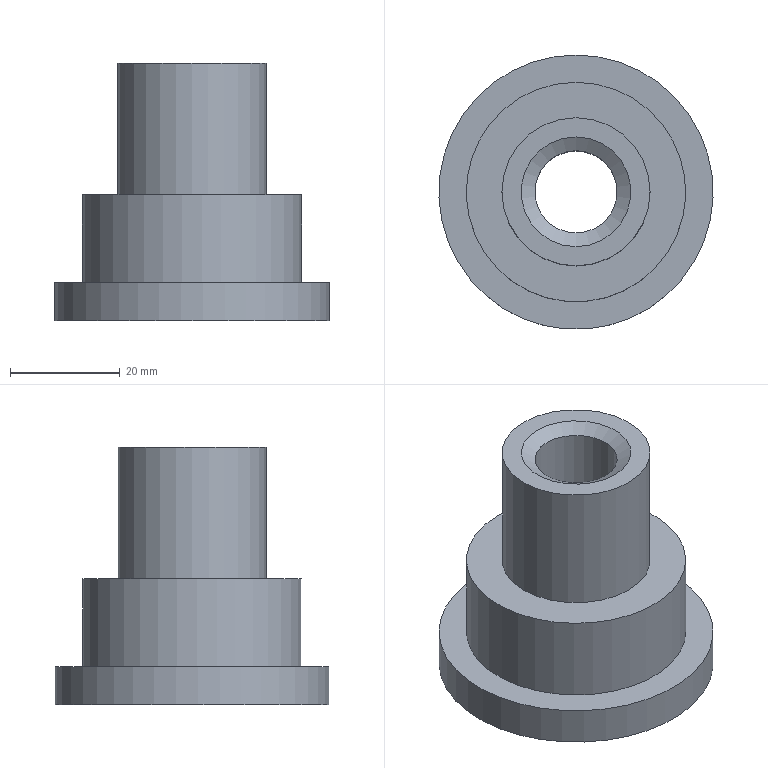Component | NX | BASE | 1 solid | 10 faces | box 50 x 50 x 47 mm | volume 38898 mm3 | cylinder 4 | plane 4 | cone 1 | torus 1 | commonest cylinder face diameters 15 x1 50 x1 40 x1 27 x1
STEP:
#1=CARTESIAN_POINT('',(0.,0.,0.));
#2=DIRECTION('',(0.,0.,1.));
#3=DIRECTION('',(1.,0.,0.));
#4=AXIS2_PLACEMENT_3D('',#1,#2,#3);
#5=CARTESIAN_POINT('',(-146.777,7.5,20.491));
#6=VERTEX_POINT('',#5);
#7=CARTESIAN_POINT('',(-146.777,0.,20.491));
#8=DIRECTION('',(0.,0.,-1.));
#9=DIRECTION('',(0.,1.,0.));
#10=AXIS2_PLACEMENT_3D('',#7,#8,#9);
#11=CIRCLE('',#10,7.5);
#12=CARTESIAN_POINT('',(-146.777,0.,22.491));
#13=DIRECTION('',(0.,0.,-1.));
#14=DIRECTION('',(0.,1.,0.));
#15=AXIS2_PLACEMENT_3D('',#12,#13,#14);
#16=CYLINDRICAL_SURFACE('',#15,7.5);
#17=CARTESIAN_POINT('',(0.,2.));
#18=DIRECTION('',(1.,0.));
#19=VECTOR('',#18,1.);
#20=LINE('',#17,#19);
#21=(GEOMETRIC_REPRESENTATION_CONTEXT(2)PARAMETRIC_REPRESENTATION_CONTEXT()REPRESENTATION_CONTEXT('',''));
#22=DEFINITIONAL_REPRESENTATION('',(#20),#21);
#23=PCURVE('',#16,#22);
#24=CARTESIAN_POINT('',(-146.777,0.,20.491));
#25=DIRECTION('',(0.,0.,-1.));
#26=DIRECTION('',(0.,1.,0.));
#27=AXIS2_PLACEMENT_3D('',#24,#25,#26);
#28=TOROIDAL_SURFACE('',#27,12.5,5.);
#29=CARTESIAN_POINT('',(0.,9.425));
#30=DIRECTION('',(1.,0.));
#31=VECTOR('',#30,1.);
#32=LINE('',#29,#31);
#33=(GEOMETRIC_REPRESENTATION_CONTEXT(2)PARAMETRIC_REPRESENTATION_CONTEXT()REPRESENTATION_CONTEXT('',''));
#34=DEFINITIONAL_REPRESENTATION('',(#32),#33);
#35=PCURVE('',#28,#34);
#36=SURFACE_CURVE('',#11,(#23,#35),.PCURVE_S1.);
#37=EDGE_CURVE('',#6,#6,#36,.T.);
#38=ORIENTED_EDGE('',*,*,#37,.F.);
#39=CARTESIAN_POINT('',(-146.777,7.5,60.991));
#40=VERTEX_POINT('',#39);
#41=CARTESIAN_POINT('',(-146.777,7.5,60.991));
#42=CARTESIAN_POINT('',(-146.777,7.5,20.491));
#43=B_SPLINE_CURVE_WITH_KNOTS('',1,(#41,#42),.UNSPECIFIED.,.F.,.F.,(2,2),(-38.5,2.),.PIECEWISE_BEZIER_KNOTS.);
#44=CARTESIAN_POINT('',(0.,0.));
#45=DIRECTION('',(0.,1.));
#46=VECTOR('',#45,1.);
#47=LINE('',#44,#46);
#48=(GEOMETRIC_REPRESENTATION_CONTEXT(2)PARAMETRIC_REPRESENTATION_CONTEXT()REPRESENTATION_CONTEXT('',''));
#49=DEFINITIONAL_REPRESENTATION('',(#47),#48);
#50=PCURVE('',#16,#49);
#51=CARTESIAN_POINT('',(6.283,0.));
#52=DIRECTION('',(0.,1.));
#53=VECTOR('',#52,1.);
#54=LINE('',#51,#53);
#55=(GEOMETRIC_REPRESENTATION_CONTEXT(2)PARAMETRIC_REPRESENTATION_CONTEXT()REPRESENTATION_CONTEXT('',''));
#56=DEFINITIONAL_REPRESENTATION('',(#54),#55);
#57=PCURVE('',#16,#56);
#58=SEAM_CURVE('',#43,(#50,#57),.PCURVE_S1.);
#59=EDGE_CURVE('',#40,#6,#58,.T.);
#60=ORIENTED_EDGE('',*,*,#59,.F.);
#61=CARTESIAN_POINT('',(-146.777,-7.5,60.991));
#62=VERTEX_POINT('',#61);
#63=CARTESIAN_POINT('',(-146.777,0.,60.991));
#64=DIRECTION('',(0.,0.,1.));
#65=DIRECTION('',(0.,-1.,0.));
#66=AXIS2_PLACEMENT_3D('',#63,#64,#65);
#67=CIRCLE('',#66,7.5);
#68=CARTESIAN_POINT('',(3.142,-38.5));
#69=DIRECTION('',(-1.,0.));
#70=VECTOR('',#69,1.);
#71=LINE('',#68,#70);
#72=(GEOMETRIC_REPRESENTATION_CONTEXT(2)PARAMETRIC_REPRESENTATION_CONTEXT()REPRESENTATION_CONTEXT('',''));
#73=DEFINITIONAL_REPRESENTATION('',(#71),#72);
#74=PCURVE('',#16,#73);
#75=CARTESIAN_POINT('',(-146.777,0.,62.491));
#76=DIRECTION('',(0.,0.,1.));
#77=DIRECTION('',(0.,-1.,0.));
#78=AXIS2_PLACEMENT_3D('',#75,#76,#77);
#79=CONICAL_SURFACE('',#78,10.,1.03);
#80=CARTESIAN_POINT('',(0.,-1.5));
#81=DIRECTION('',(1.,0.));
#82=VECTOR('',#81,1.);
#83=LINE('',#80,#82);
#84=(GEOMETRIC_REPRESENTATION_CONTEXT(2)PARAMETRIC_REPRESENTATION_CONTEXT()REPRESENTATION_CONTEXT('',''));
#85=DEFINITIONAL_REPRESENTATION('',(#83),#84);
#86=PCURVE('',#79,#85);
#87=SURFACE_CURVE('',#67,(#74,#86),.PCURVE_S1.);
#88=EDGE_CURVE('',#62,#40,#87,.T.);
#89=ORIENTED_EDGE('',*,*,#88,.F.);
#90=CARTESIAN_POINT('',(-146.777,0.,60.991));
#91=DIRECTION('',(0.,0.,1.));
#92=DIRECTION('',(0.,-1.,0.));
#93=AXIS2_PLACEMENT_3D('',#90,#91,#92);
#94=CIRCLE('',#93,7.5);
#95=CARTESIAN_POINT('',(9.425,-38.5));
#96=DIRECTION('',(-1.,0.));
#97=VECTOR('',#96,1.);
#98=LINE('',#95,#97);
#99=(GEOMETRIC_REPRESENTATION_CONTEXT(2)PARAMETRIC_REPRESENTATION_CONTEXT()REPRESENTATION_CONTEXT('',''));
#100=DEFINITIONAL_REPRESENTATION('',(#98),#99);
#101=PCURVE('',#16,#100);
#102=CARTESIAN_POINT('',(0.,-1.5));
#103=DIRECTION('',(1.,0.));
#104=VECTOR('',#103,1.);
#105=LINE('',#102,#104);
#106=(GEOMETRIC_REPRESENTATION_CONTEXT(2)PARAMETRIC_REPRESENTATION_CONTEXT()REPRESENTATION_CONTEXT('',''));
#107=DEFINITIONAL_REPRESENTATION('',(#105),#106);
#108=PCURVE('',#79,#107);
#109=SURFACE_CURVE('',#94,(#101,#108),.PCURVE_S1.);
#110=EDGE_CURVE('',#40,#62,#109,.T.);
#111=ORIENTED_EDGE('',*,*,#110,.F.);
#112=ORIENTED_EDGE('',*,*,#59,.T.);
#113=EDGE_LOOP('',(#38,#60,#89,#111,#112));
#114=FACE_BOUND('',#113,.F.);
#115=ADVANCED_FACE('',(#114),#16,.F.);
#116=CARTESIAN_POINT('',(-146.777,12.5,15.491));
#117=VERTEX_POINT('',#116);
#118=CARTESIAN_POINT('',(-146.777,0.,15.491));
#119=DIRECTION('',(0.,0.,1.));
#120=DIRECTION('',(0.,1.,0.));
#121=AXIS2_PLACEMENT_3D('',#118,#119,#120);
#122=CIRCLE('',#121,12.5);
#123=CARTESIAN_POINT('',(-139.277,0.,15.491));
#124=DIRECTION('',(0.,0.,-1.));
#125=DIRECTION('',(0.,1.,0.));
#126=AXIS2_PLACEMENT_3D('',#123,#124,#125);
#127=PLANE('',#126);
#128=CARTESIAN_POINT('',(12.5,-7.5));
#129=CARTESIAN_POINT('',(12.5,-29.151));
#130=CARTESIAN_POINT('',(-6.25,-18.325));
#131=CARTESIAN_POINT('',(-25.,-7.5));
#132=CARTESIAN_POINT('',(-6.25,3.325));
#133=CARTESIAN_POINT('',(12.5,14.151));
#134=CARTESIAN_POINT('',(12.5,-7.5));
#135=(BOUNDED_CURVE()B_SPLINE_CURVE(2,(#128,#129,#130,#131,#132,#133,#134),.UNSPECIFIED.,.T.,.F.)B_SPLINE_CURVE_WITH_KNOTS((1,2,2,2,2,1),(-2.094,0.,2.094,4.189,6.283,8.378),.UNSPECIFIED.)CURVE()GEOMETRIC_REPRESENTATION_ITEM()RATIONAL_B_SPLINE_CURVE((1.,0.5,1.,0.5,1.,0.5,1.))REPRESENTATION_ITEM(''));
#136=(GEOMETRIC_REPRESENTATION_CONTEXT(2)PARAMETRIC_REPRESENTATION_CONTEXT()REPRESENTATION_CONTEXT('',''));
#137=DEFINITIONAL_REPRESENTATION('',(#135),#136);
#138=PCURVE('',#127,#137);
#139=CARTESIAN_POINT('',(6.283,7.854));
#140=DIRECTION('',(-1.,0.));
#141=VECTOR('',#140,1.);
#142=LINE('',#139,#141);
#143=(GEOMETRIC_REPRESENTATION_CONTEXT(2)PARAMETRIC_REPRESENTATION_CONTEXT()REPRESENTATION_CONTEXT('',''));
#144=DEFINITIONAL_REPRESENTATION('',(#142),#143);
#145=PCURVE('',#28,#144);
#146=SURFACE_CURVE('',#122,(#138,#145),.PCURVE_S1.);
#147=EDGE_CURVE('',#117,#117,#146,.T.);
#148=ORIENTED_EDGE('',*,*,#147,.T.);
#149=EDGE_LOOP('',(#148));
#150=FACE_BOUND('',#149,.T.);
#151=CARTESIAN_POINT('',(-146.777,25.,15.491));
#152=VERTEX_POINT('',#151);
#153=CARTESIAN_POINT('',(-146.777,0.,15.491));
#154=DIRECTION('',(0.,0.,-1.));
#155=DIRECTION('',(0.,1.,0.));
#156=AXIS2_PLACEMENT_3D('',#153,#154,#155);
#157=CIRCLE('',#156,25.);
#158=CARTESIAN_POINT('',(0.,-7.5));
#159=DIRECTION('',(1.,0.));
#160=AXIS2_PLACEMENT_2D('',#158,#159);
#161=CIRCLE('',#160,25.);
#162=(GEOMETRIC_REPRESENTATION_CONTEXT(2)PARAMETRIC_REPRESENTATION_CONTEXT()REPRESENTATION_CONTEXT('',''));
#163=DEFINITIONAL_REPRESENTATION('',(#161),#162);
#164=PCURVE('',#127,#163);
#165=CARTESIAN_POINT('',(-146.777,0.,22.491));
#166=DIRECTION('',(0.,0.,-1.));
#167=DIRECTION('',(0.,1.,0.));
#168=AXIS2_PLACEMENT_3D('',#165,#166,#167);
#169=CYLINDRICAL_SURFACE('',#168,25.);
#170=CARTESIAN_POINT('',(0.,7.));
#171=DIRECTION('',(1.,0.));
#172=VECTOR('',#171,1.);
#173=LINE('',#170,#172);
#174=(GEOMETRIC_REPRESENTATION_CONTEXT(2)PARAMETRIC_REPRESENTATION_CONTEXT()REPRESENTATION_CONTEXT('',''));
#175=DEFINITIONAL_REPRESENTATION('',(#173),#174);
#176=PCURVE('',#169,#175);
#177=SURFACE_CURVE('',#157,(#164,#176),.PCURVE_S1.);
#178=EDGE_CURVE('',#152,#152,#177,.T.);
#179=ORIENTED_EDGE('',*,*,#178,.T.);
#180=EDGE_LOOP('',(#179));
#181=FACE_BOUND('',#180,.T.);
#182=ADVANCED_FACE('',(#150,#181),#127,.T.);
#183=CARTESIAN_POINT('',(-146.777,25.,22.491));
#184=VERTEX_POINT('',#183);
#185=CARTESIAN_POINT('',(-146.777,0.,22.491));
#186=DIRECTION('',(0.,0.,-1.));
#187=DIRECTION('',(0.,1.,0.));
#188=AXIS2_PLACEMENT_3D('',#185,#186,#187);
#189=CIRCLE('',#188,25.);
#190=CARTESIAN_POINT('',(0.,0.));
#191=DIRECTION('',(1.,0.));
#192=VECTOR('',#191,1.);
#193=LINE('',#190,#192);
#194=(GEOMETRIC_REPRESENTATION_CONTEXT(2)PARAMETRIC_REPRESENTATION_CONTEXT()REPRESENTATION_CONTEXT('',''));
#195=DEFINITIONAL_REPRESENTATION('',(#193),#194);
#196=PCURVE('',#169,#195);
#197=CARTESIAN_POINT('',(-121.777,0.,22.491));
#198=DIRECTION('',(0.,0.,1.));
#199=DIRECTION('',(0.,-1.,0.));
#200=AXIS2_PLACEMENT_3D('',#197,#198,#199);
#201=PLANE('',#200);
#202=CARTESIAN_POINT('',(-25.,-25.));
#203=CARTESIAN_POINT('',(-25.,18.301));
#204=CARTESIAN_POINT('',(12.5,-3.349));
#205=CARTESIAN_POINT('',(50.,-25.));
#206=CARTESIAN_POINT('',(12.5,-46.651));
#207=CARTESIAN_POINT('',(-25.,-68.301));
#208=CARTESIAN_POINT('',(-25.,-25.));
#209=(BOUNDED_CURVE()B_SPLINE_CURVE(2,(#202,#203,#204,#205,#206,#207,#208),.UNSPECIFIED.,.T.,.F.)B_SPLINE_CURVE_WITH_KNOTS((1,2,2,2,2,1),(-2.094,0.,2.094,4.189,6.283,8.378),.UNSPECIFIED.)CURVE()GEOMETRIC_REPRESENTATION_ITEM()RATIONAL_B_SPLINE_CURVE((1.,0.5,1.,0.5,1.,0.5,1.))REPRESENTATION_ITEM(''));
#210=(GEOMETRIC_REPRESENTATION_CONTEXT(2)PARAMETRIC_REPRESENTATION_CONTEXT()REPRESENTATION_CONTEXT('',''));
#211=DEFINITIONAL_REPRESENTATION('',(#209),#210);
#212=PCURVE('',#201,#211);
#213=SURFACE_CURVE('',#189,(#196,#212),.PCURVE_S1.);
#214=EDGE_CURVE('',#184,#184,#213,.T.);
#215=ORIENTED_EDGE('',*,*,#214,.T.);
#216=CARTESIAN_POINT('',(-146.777,25.,22.491));
#217=CARTESIAN_POINT('',(-146.777,25.,15.491));
#218=B_SPLINE_CURVE_WITH_KNOTS('',1,(#216,#217),.UNSPECIFIED.,.F.,.F.,(2,2),(0.,7.),.PIECEWISE_BEZIER_KNOTS.);
#219=CARTESIAN_POINT('',(6.283,0.));
#220=DIRECTION('',(0.,1.));
#221=VECTOR('',#220,1.);
#222=LINE('',#219,#221);
#223=(GEOMETRIC_REPRESENTATION_CONTEXT(2)PARAMETRIC_REPRESENTATION_CONTEXT()REPRESENTATION_CONTEXT('',''));
#224=DEFINITIONAL_REPRESENTATION('',(#222),#223);
#225=PCURVE('',#169,#224);
#226=CARTESIAN_POINT('',(0.,0.));
#227=DIRECTION('',(0.,1.));
#228=VECTOR('',#227,1.);
#229=LINE('',#226,#228);
#230=(GEOMETRIC_REPRESENTATION_CONTEXT(2)PARAMETRIC_REPRESENTATION_CONTEXT()REPRESENTATION_CONTEXT('',''));
#231=DEFINITIONAL_REPRESENTATION('',(#229),#230);
#232=PCURVE('',#169,#231);
#233=SEAM_CURVE('',#218,(#225,#232),.PCURVE_S1.);
#234=EDGE_CURVE('',#184,#152,#233,.T.);
#235=ORIENTED_EDGE('',*,*,#234,.T.);
#236=ORIENTED_EDGE('',*,*,#178,.F.);
#237=ORIENTED_EDGE('',*,*,#234,.F.);
#238=EDGE_LOOP('',(#215,#235,#236,#237));
#239=FACE_BOUND('',#238,.T.);
#240=ADVANCED_FACE('',(#239),#169,.T.);
#241=CARTESIAN_POINT('',(-146.777,20.,22.491));
#242=VERTEX_POINT('',#241);
#243=CARTESIAN_POINT('',(-146.777,0.,22.491));
#244=DIRECTION('',(0.,0.,-1.));
#245=DIRECTION('',(0.,1.,0.));
#246=AXIS2_PLACEMENT_3D('',#243,#244,#245);
#247=CIRCLE('',#246,20.);
#248=CARTESIAN_POINT('',(-20.,-25.));
#249=CARTESIAN_POINT('',(-20.,9.641));
#250=CARTESIAN_POINT('',(10.,-7.679));
#251=CARTESIAN_POINT('',(40.,-25.));
#252=CARTESIAN_POINT('',(10.,-42.321));
#253=CARTESIAN_POINT('',(-20.,-59.641));
#254=CARTESIAN_POINT('',(-20.,-25.));
#255=(BOUNDED_CURVE()B_SPLINE_CURVE(2,(#248,#249,#250,#251,#252,#253,#254),.UNSPECIFIED.,.T.,.F.)B_SPLINE_CURVE_WITH_KNOTS((1,2,2,2,2,1),(-2.094,0.,2.094,4.189,6.283,8.378),.UNSPECIFIED.)CURVE()GEOMETRIC_REPRESENTATION_ITEM()RATIONAL_B_SPLINE_CURVE((1.,0.5,1.,0.5,1.,0.5,1.))REPRESENTATION_ITEM(''));
#256=(GEOMETRIC_REPRESENTATION_CONTEXT(2)PARAMETRIC_REPRESENTATION_CONTEXT()REPRESENTATION_CONTEXT('',''));
#257=DEFINITIONAL_REPRESENTATION('',(#255),#256);
#258=PCURVE('',#201,#257);
#259=CARTESIAN_POINT('',(-146.777,0.,22.491));
#260=DIRECTION('',(0.,0.,-1.));
#261=DIRECTION('',(0.,1.,0.));
#262=AXIS2_PLACEMENT_3D('',#259,#260,#261);
#263=CYLINDRICAL_SURFACE('',#262,20.);
#264=CARTESIAN_POINT('',(0.,0.));
#265=DIRECTION('',(1.,0.));
#266=VECTOR('',#265,1.);
#267=LINE('',#264,#266);
#268=(GEOMETRIC_REPRESENTATION_CONTEXT(2)PARAMETRIC_REPRESENTATION_CONTEXT()REPRESENTATION_CONTEXT('',''));
#269=DEFINITIONAL_REPRESENTATION('',(#267),#268);
#270=PCURVE('',#263,#269);
#271=SURFACE_CURVE('',#247,(#258,#270),.PCURVE_S1.);
#272=EDGE_CURVE('',#242,#242,#271,.T.);
#273=ORIENTED_EDGE('',*,*,#272,.T.);
#274=EDGE_LOOP('',(#273));
#275=FACE_BOUND('',#274,.T.);
#276=ORIENTED_EDGE('',*,*,#214,.F.);
#277=EDGE_LOOP('',(#276));
#278=FACE_BOUND('',#277,.T.);
#279=ADVANCED_FACE('',(#275,#278),#201,.T.);
#280=CARTESIAN_POINT('',(-146.777,20.,38.491));
#281=VERTEX_POINT('',#280);
#282=CARTESIAN_POINT('',(-146.777,0.,38.491));
#283=DIRECTION('',(0.,0.,-1.));
#284=DIRECTION('',(0.,1.,0.));
#285=AXIS2_PLACEMENT_3D('',#282,#283,#284);
#286=CIRCLE('',#285,20.);
#287=CARTESIAN_POINT('',(0.,-16.));
#288=DIRECTION('',(1.,0.));
#289=VECTOR('',#288,1.);
#290=LINE('',#287,#289);
#291=(GEOMETRIC_REPRESENTATION_CONTEXT(2)PARAMETRIC_REPRESENTATION_CONTEXT()REPRESENTATION_CONTEXT('',''));
#292=DEFINITIONAL_REPRESENTATION('',(#290),#291);
#293=PCURVE('',#263,#292);
#294=CARTESIAN_POINT('',(-126.777,0.,38.491));
#295=DIRECTION('',(0.,0.,1.));
#296=DIRECTION('',(0.,-1.,0.));
#297=AXIS2_PLACEMENT_3D('',#294,#295,#296);
#298=PLANE('',#297);
#299=CARTESIAN_POINT('',(-20.,-20.));
#300=CARTESIAN_POINT('',(-20.,14.641));
#301=CARTESIAN_POINT('',(10.,-2.679));
#302=CARTESIAN_POINT('',(40.,-20.));
#303=CARTESIAN_POINT('',(10.,-37.321));
#304=CARTESIAN_POINT('',(-20.,-54.641));
#305=CARTESIAN_POINT('',(-20.,-20.));
#306=(BOUNDED_CURVE()B_SPLINE_CURVE(2,(#299,#300,#301,#302,#303,#304,#305),.UNSPECIFIED.,.T.,.F.)B_SPLINE_CURVE_WITH_KNOTS((1,2,2,2,2,1),(-2.094,0.,2.094,4.189,6.283,8.378),.UNSPECIFIED.)CURVE()GEOMETRIC_REPRESENTATION_ITEM()RATIONAL_B_SPLINE_CURVE((1.,0.5,1.,0.5,1.,0.5,1.))REPRESENTATION_ITEM(''));
#307=(GEOMETRIC_REPRESENTATION_CONTEXT(2)PARAMETRIC_REPRESENTATION_CONTEXT()REPRESENTATION_CONTEXT('',''));
#308=DEFINITIONAL_REPRESENTATION('',(#306),#307);
#309=PCURVE('',#298,#308);
#310=SURFACE_CURVE('',#286,(#293,#309),.PCURVE_S1.);
#311=EDGE_CURVE('',#281,#281,#310,.T.);
#312=ORIENTED_EDGE('',*,*,#311,.T.);
#313=CARTESIAN_POINT('',(-146.777,20.,38.491));
#314=CARTESIAN_POINT('',(-146.777,20.,22.491));
#315=B_SPLINE_CURVE_WITH_KNOTS('',1,(#313,#314),.UNSPECIFIED.,.F.,.F.,(2,2),(-16.,0.),.PIECEWISE_BEZIER_KNOTS.);
#316=CARTESIAN_POINT('',(6.283,0.));
#317=DIRECTION('',(0.,1.));
#318=VECTOR('',#317,1.);
#319=LINE('',#316,#318);
#320=(GEOMETRIC_REPRESENTATION_CONTEXT(2)PARAMETRIC_REPRESENTATION_CONTEXT()REPRESENTATION_CONTEXT('',''));
#321=DEFINITIONAL_REPRESENTATION('',(#319),#320);
#322=PCURVE('',#263,#321);
#323=CARTESIAN_POINT('',(0.,0.));
#324=DIRECTION('',(0.,1.));
#325=VECTOR('',#324,1.);
#326=LINE('',#323,#325);
#327=(GEOMETRIC_REPRESENTATION_CONTEXT(2)PARAMETRIC_REPRESENTATION_CONTEXT()REPRESENTATION_CONTEXT('',''));
#328=DEFINITIONAL_REPRESENTATION('',(#326),#327);
#329=PCURVE('',#263,#328);
#330=SEAM_CURVE('',#315,(#322,#329),.PCURVE_S1.);
#331=EDGE_CURVE('',#281,#242,#330,.T.);
#332=ORIENTED_EDGE('',*,*,#331,.T.);
#333=ORIENTED_EDGE('',*,*,#272,.F.);
#334=ORIENTED_EDGE('',*,*,#331,.F.);
#335=EDGE_LOOP('',(#312,#332,#333,#334));
#336=FACE_BOUND('',#335,.T.);
#337=ADVANCED_FACE('',(#336),#263,.T.);
#338=CARTESIAN_POINT('',(-146.777,13.5,38.491));
#339=VERTEX_POINT('',#338);
#340=CARTESIAN_POINT('',(-146.777,0.,38.491));
#341=DIRECTION('',(0.,0.,-1.));
#342=DIRECTION('',(0.,1.,0.));
#343=AXIS2_PLACEMENT_3D('',#340,#341,#342);
#344=CIRCLE('',#343,13.5);
#345=CARTESIAN_POINT('',(-13.5,-20.));
#346=CARTESIAN_POINT('',(-13.5,3.383));
#347=CARTESIAN_POINT('',(6.75,-8.309));
#348=CARTESIAN_POINT('',(27.,-20.));
#349=CARTESIAN_POINT('',(6.75,-31.691));
#350=CARTESIAN_POINT('',(-13.5,-43.383));
#351=CARTESIAN_POINT('',(-13.5,-20.));
#352=(BOUNDED_CURVE()B_SPLINE_CURVE(2,(#345,#346,#347,#348,#349,#350,#351),.UNSPECIFIED.,.T.,.F.)B_SPLINE_CURVE_WITH_KNOTS((1,2,2,2,2,1),(-2.094,0.,2.094,4.189,6.283,8.378),.UNSPECIFIED.)CURVE()GEOMETRIC_REPRESENTATION_ITEM()RATIONAL_B_SPLINE_CURVE((1.,0.5,1.,0.5,1.,0.5,1.))REPRESENTATION_ITEM(''));
#353=(GEOMETRIC_REPRESENTATION_CONTEXT(2)PARAMETRIC_REPRESENTATION_CONTEXT()REPRESENTATION_CONTEXT('',''));
#354=DEFINITIONAL_REPRESENTATION('',(#352),#353);
#355=PCURVE('',#298,#354);
#356=CARTESIAN_POINT('',(-146.777,0.,22.491));
#357=DIRECTION('',(0.,0.,-1.));
#358=DIRECTION('',(0.,1.,0.));
#359=AXIS2_PLACEMENT_3D('',#356,#357,#358);
#360=CYLINDRICAL_SURFACE('',#359,13.5);
#361=CARTESIAN_POINT('',(0.,-16.));
#362=DIRECTION('',(1.,0.));
#363=VECTOR('',#362,1.);
#364=LINE('',#361,#363);
#365=(GEOMETRIC_REPRESENTATION_CONTEXT(2)PARAMETRIC_REPRESENTATION_CONTEXT()REPRESENTATION_CONTEXT('',''));
#366=DEFINITIONAL_REPRESENTATION('',(#364),#365);
#367=PCURVE('',#360,#366);
#368=SURFACE_CURVE('',#344,(#355,#367),.PCURVE_S1.);
#369=EDGE_CURVE('',#339,#339,#368,.T.);
#370=ORIENTED_EDGE('',*,*,#369,.T.);
#371=EDGE_LOOP('',(#370));
#372=FACE_BOUND('',#371,.T.);
#373=ORIENTED_EDGE('',*,*,#311,.F.);
#374=EDGE_LOOP('',(#373));
#375=FACE_BOUND('',#374,.T.);
#376=ADVANCED_FACE('',(#372,#375),#298,.T.);
#377=CARTESIAN_POINT('',(-146.777,13.5,62.491));
#378=VERTEX_POINT('',#377);
#379=CARTESIAN_POINT('',(-146.777,0.,62.491));
#380=DIRECTION('',(0.,0.,-1.));
#381=DIRECTION('',(0.,1.,0.));
#382=AXIS2_PLACEMENT_3D('',#379,#380,#381);
#383=CIRCLE('',#382,13.5);
#384=CARTESIAN_POINT('',(0.,-40.));
#385=DIRECTION('',(1.,0.));
#386=VECTOR('',#385,1.);
#387=LINE('',#384,#386);
#388=(GEOMETRIC_REPRESENTATION_CONTEXT(2)PARAMETRIC_REPRESENTATION_CONTEXT()REPRESENTATION_CONTEXT('',''));
#389=DEFINITIONAL_REPRESENTATION('',(#387),#388);
#390=PCURVE('',#360,#389);
#391=CARTESIAN_POINT('',(-133.277,0.,62.491));
#392=DIRECTION('',(0.,0.,1.));
#393=DIRECTION('',(0.,-1.,0.));
#394=AXIS2_PLACEMENT_3D('',#391,#392,#393);
#395=PLANE('',#394);
#396=CARTESIAN_POINT('',(-13.5,-13.5));
#397=CARTESIAN_POINT('',(-13.5,9.883));
#398=CARTESIAN_POINT('',(6.75,-1.809));
#399=CARTESIAN_POINT('',(27.,-13.5));
#400=CARTESIAN_POINT('',(6.75,-25.191));
#401=CARTESIAN_POINT('',(-13.5,-36.883));
#402=CARTESIAN_POINT('',(-13.5,-13.5));
#403=(BOUNDED_CURVE()B_SPLINE_CURVE(2,(#396,#397,#398,#399,#400,#401,#402),.UNSPECIFIED.,.T.,.F.)B_SPLINE_CURVE_WITH_KNOTS((1,2,2,2,2,1),(-2.094,0.,2.094,4.189,6.283,8.378),.UNSPECIFIED.)CURVE()GEOMETRIC_REPRESENTATION_ITEM()RATIONAL_B_SPLINE_CURVE((1.,0.5,1.,0.5,1.,0.5,1.))REPRESENTATION_ITEM(''));
#404=(GEOMETRIC_REPRESENTATION_CONTEXT(2)PARAMETRIC_REPRESENTATION_CONTEXT()REPRESENTATION_CONTEXT('',''));
#405=DEFINITIONAL_REPRESENTATION('',(#403),#404);
#406=PCURVE('',#395,#405);
#407=SURFACE_CURVE('',#383,(#390,#406),.PCURVE_S1.);
#408=EDGE_CURVE('',#378,#378,#407,.T.);
#409=ORIENTED_EDGE('',*,*,#408,.T.);
#410=CARTESIAN_POINT('',(-146.777,13.5,62.491));
#411=CARTESIAN_POINT('',(-146.777,13.5,38.491));
#412=B_SPLINE_CURVE_WITH_KNOTS('',1,(#410,#411),.UNSPECIFIED.,.F.,.F.,(2,2),(-40.,-16.),.PIECEWISE_BEZIER_KNOTS.);
#413=CARTESIAN_POINT('',(6.283,0.));
#414=DIRECTION('',(0.,1.));
#415=VECTOR('',#414,1.);
#416=LINE('',#413,#415);
#417=(GEOMETRIC_REPRESENTATION_CONTEXT(2)PARAMETRIC_REPRESENTATION_CONTEXT()REPRESENTATION_CONTEXT('',''));
#418=DEFINITIONAL_REPRESENTATION('',(#416),#417);
#419=PCURVE('',#360,#418);
#420=CARTESIAN_POINT('',(0.,0.));
#421=DIRECTION('',(0.,1.));
#422=VECTOR('',#421,1.);
#423=LINE('',#420,#422);
#424=(GEOMETRIC_REPRESENTATION_CONTEXT(2)PARAMETRIC_REPRESENTATION_CONTEXT()REPRESENTATION_CONTEXT('',''));
#425=DEFINITIONAL_REPRESENTATION('',(#423),#424);
#426=PCURVE('',#360,#425);
#427=SEAM_CURVE('',#412,(#419,#426),.PCURVE_S1.);
#428=EDGE_CURVE('',#378,#339,#427,.T.);
#429=ORIENTED_EDGE('',*,*,#428,.T.);
#430=ORIENTED_EDGE('',*,*,#369,.F.);
#431=ORIENTED_EDGE('',*,*,#428,.F.);
#432=EDGE_LOOP('',(#409,#429,#430,#431));
#433=FACE_BOUND('',#432,.T.);
#434=ADVANCED_FACE('',(#433),#360,.T.);
#435=CARTESIAN_POINT('',(-146.777,-10.,62.491));
#436=VERTEX_POINT('',#435);
#437=CARTESIAN_POINT('',(-146.777,0.,62.491));
#438=DIRECTION('',(0.,0.,-1.));
#439=DIRECTION('',(0.,-1.,0.));
#440=AXIS2_PLACEMENT_3D('',#437,#438,#439);
#441=CIRCLE('',#440,10.);
#442=CARTESIAN_POINT('',(10.,-13.5));
#443=CARTESIAN_POINT('',(10.,-30.821));
#444=CARTESIAN_POINT('',(-5.,-22.16));
#445=CARTESIAN_POINT('',(-20.,-13.5));
#446=CARTESIAN_POINT('',(-5.,-4.84));
#447=CARTESIAN_POINT('',(10.,3.821));
#448=CARTESIAN_POINT('',(10.,-13.5));
#449=(BOUNDED_CURVE()B_SPLINE_CURVE(2,(#442,#443,#444,#445,#446,#447,#448),.UNSPECIFIED.,.T.,.F.)B_SPLINE_CURVE_WITH_KNOTS((1,2,2,2,2,1),(-2.094,0.,2.094,4.189,6.283,8.378),.UNSPECIFIED.)CURVE()GEOMETRIC_REPRESENTATION_ITEM()RATIONAL_B_SPLINE_CURVE((1.,0.5,1.,0.5,1.,0.5,1.))REPRESENTATION_ITEM(''));
#450=(GEOMETRIC_REPRESENTATION_CONTEXT(2)PARAMETRIC_REPRESENTATION_CONTEXT()REPRESENTATION_CONTEXT('',''));
#451=DEFINITIONAL_REPRESENTATION('',(#449),#450);
#452=PCURVE('',#395,#451);
#453=CARTESIAN_POINT('',(6.283,0.));
#454=DIRECTION('',(-1.,0.));
#455=VECTOR('',#454,1.);
#456=LINE('',#453,#455);
#457=(GEOMETRIC_REPRESENTATION_CONTEXT(2)PARAMETRIC_REPRESENTATION_CONTEXT()REPRESENTATION_CONTEXT('',''));
#458=DEFINITIONAL_REPRESENTATION('',(#456),#457);
#459=PCURVE('',#79,#458);
#460=SURFACE_CURVE('',#441,(#452,#459),.PCURVE_S1.);
#461=EDGE_CURVE('',#436,#436,#460,.T.);
#462=ORIENTED_EDGE('',*,*,#461,.T.);
#463=EDGE_LOOP('',(#462));
#464=FACE_BOUND('',#463,.T.);
#465=ORIENTED_EDGE('',*,*,#408,.F.);
#466=EDGE_LOOP('',(#465));
#467=FACE_BOUND('',#466,.T.);
#468=ADVANCED_FACE('',(#464,#467),#395,.T.);
#469=ORIENTED_EDGE('',*,*,#110,.T.);
#470=CARTESIAN_POINT('',(-146.777,-7.5,60.991));
#471=CARTESIAN_POINT('',(-146.777,-10.,62.491));
#472=B_SPLINE_CURVE_WITH_KNOTS('',1,(#470,#471),.UNSPECIFIED.,.F.,.F.,(2,2),(-2.915,0.),.PIECEWISE_BEZIER_KNOTS.);
#473=CARTESIAN_POINT('',(6.283,0.));
#474=DIRECTION('',(0.,1.));
#475=VECTOR('',#474,1.);
#476=LINE('',#473,#475);
#477=(GEOMETRIC_REPRESENTATION_CONTEXT(2)PARAMETRIC_REPRESENTATION_CONTEXT()REPRESENTATION_CONTEXT('',''));
#478=DEFINITIONAL_REPRESENTATION('',(#476),#477);
#479=PCURVE('',#79,#478);
#480=CARTESIAN_POINT('',(0.,0.));
#481=DIRECTION('',(0.,1.));
#482=VECTOR('',#481,1.);
#483=LINE('',#480,#482);
#484=(GEOMETRIC_REPRESENTATION_CONTEXT(2)PARAMETRIC_REPRESENTATION_CONTEXT()REPRESENTATION_CONTEXT('',''));
#485=DEFINITIONAL_REPRESENTATION('',(#483),#484);
#486=PCURVE('',#79,#485);
#487=SEAM_CURVE('',#472,(#479,#486),.PCURVE_S1.);
#488=EDGE_CURVE('',#62,#436,#487,.T.);
#489=ORIENTED_EDGE('',*,*,#488,.T.);
#490=ORIENTED_EDGE('',*,*,#461,.T.);
#491=ORIENTED_EDGE('',*,*,#488,.F.);
#492=ORIENTED_EDGE('',*,*,#88,.T.);
#493=EDGE_LOOP('',(#469,#489,#490,#491,#492));
#494=FACE_BOUND('',#493,.F.);
#495=ADVANCED_FACE('',(#494),#79,.F.);
#496=ORIENTED_EDGE('',*,*,#147,.F.);
#497=CARTESIAN_POINT('',(-146.777,12.5,15.491));
#498=CARTESIAN_POINT('',(-146.777,11.163,15.491));
#499=CARTESIAN_POINT('',(-146.777,9.861,15.916));
#500=CARTESIAN_POINT('',(-146.777,8.74,16.732));
#501=CARTESIAN_POINT('',(-146.777,7.925,17.853));
#502=CARTESIAN_POINT('',(-146.777,7.5,19.155));
#503=CARTESIAN_POINT('',(-146.777,7.5,20.491));
#504=(BOUNDED_CURVE()B_SPLINE_CURVE(6,(#497,#498,#499,#500,#501,#502,#503),.UNSPECIFIED.,.F.,.F.)B_SPLINE_CURVE_WITH_KNOTS((7,7),(1.571,3.142),.PIECEWISE_BEZIER_KNOTS.)CURVE()GEOMETRIC_REPRESENTATION_ITEM()RATIONAL_B_SPLINE_CURVE((1.031,1.01,0.9979,0.994,0.9979,1.01,1.031))REPRESENTATION_ITEM(''));
#505=CARTESIAN_POINT('',(6.283,6.283));
#506=DIRECTION('',(0.,1.));
#507=VECTOR('',#506,1.);
#508=LINE('',#505,#507);
#509=(GEOMETRIC_REPRESENTATION_CONTEXT(2)PARAMETRIC_REPRESENTATION_CONTEXT()REPRESENTATION_CONTEXT('',''));
#510=DEFINITIONAL_REPRESENTATION('',(#508),#509);
#511=PCURVE('',#28,#510);
#512=CARTESIAN_POINT('',(0.,6.283));
#513=DIRECTION('',(0.,1.));
#514=VECTOR('',#513,1.);
#515=LINE('',#512,#514);
#516=(GEOMETRIC_REPRESENTATION_CONTEXT(2)PARAMETRIC_REPRESENTATION_CONTEXT()REPRESENTATION_CONTEXT('',''));
#517=DEFINITIONAL_REPRESENTATION('',(#515),#516);
#518=PCURVE('',#28,#517);
#519=SEAM_CURVE('',#504,(#511,#518),.PCURVE_S1.);
#520=EDGE_CURVE('',#117,#6,#519,.T.);
#521=ORIENTED_EDGE('',*,*,#520,.T.);
#522=ORIENTED_EDGE('',*,*,#37,.F.);
#523=ORIENTED_EDGE('',*,*,#520,.F.);
#524=EDGE_LOOP('',(#496,#521,#522,#523));
#525=FACE_BOUND('',#524,.T.);
#526=ADVANCED_FACE('',(#525),#28,.T.);
#527=CLOSED_SHELL('',(#115,#182,#240,#279,#337,#376,#434,#468,#495,#526));
#528=MANIFOLD_SOLID_BREP('',#527);
#529=(LENGTH_UNIT()NAMED_UNIT(*)SI_UNIT(.MILLI.,.METRE.));
#530=UNCERTAINTY_MEASURE_WITH_UNIT(LENGTH_MEASURE(0.00001),#529,'','');
#531=(NAMED_UNIT(*)PLANE_ANGLE_UNIT()SI_UNIT($,.RADIAN.));
#532=(NAMED_UNIT(*)SI_UNIT($,.STERADIAN.)SOLID_ANGLE_UNIT());
#533=(GEOMETRIC_REPRESENTATION_CONTEXT(3)GLOBAL_UNCERTAINTY_ASSIGNED_CONTEXT((#530))GLOBAL_UNIT_ASSIGNED_CONTEXT((#529,#531,#532))REPRESENTATION_CONTEXT('',''));
#534=ADVANCED_BREP_SHAPE_REPRESENTATION('',(#4,#528),#533);